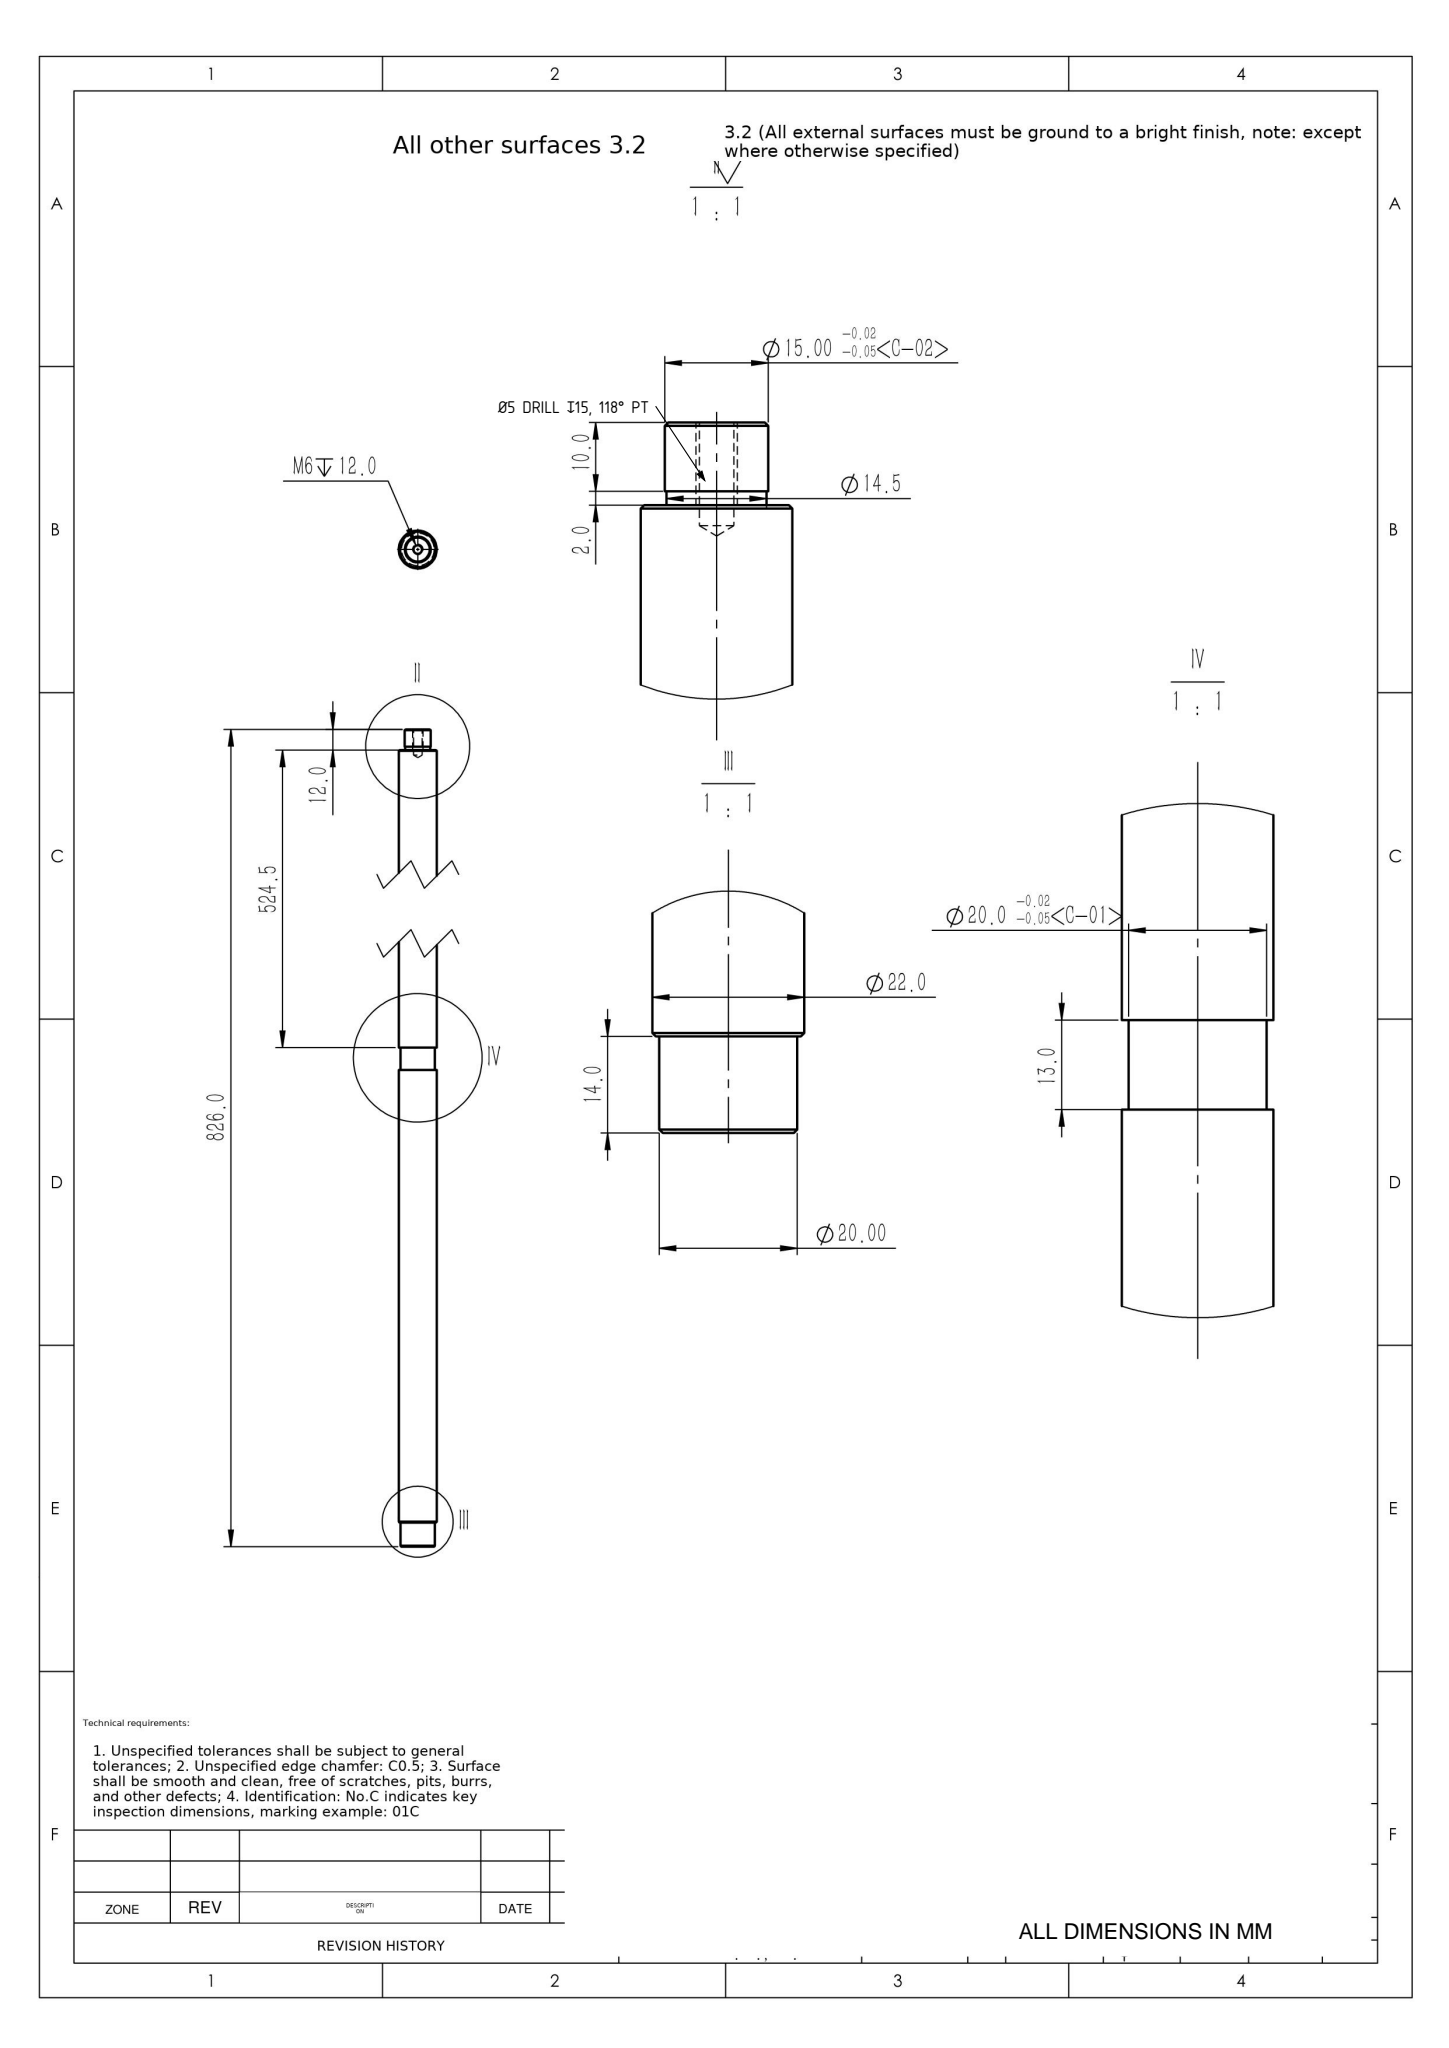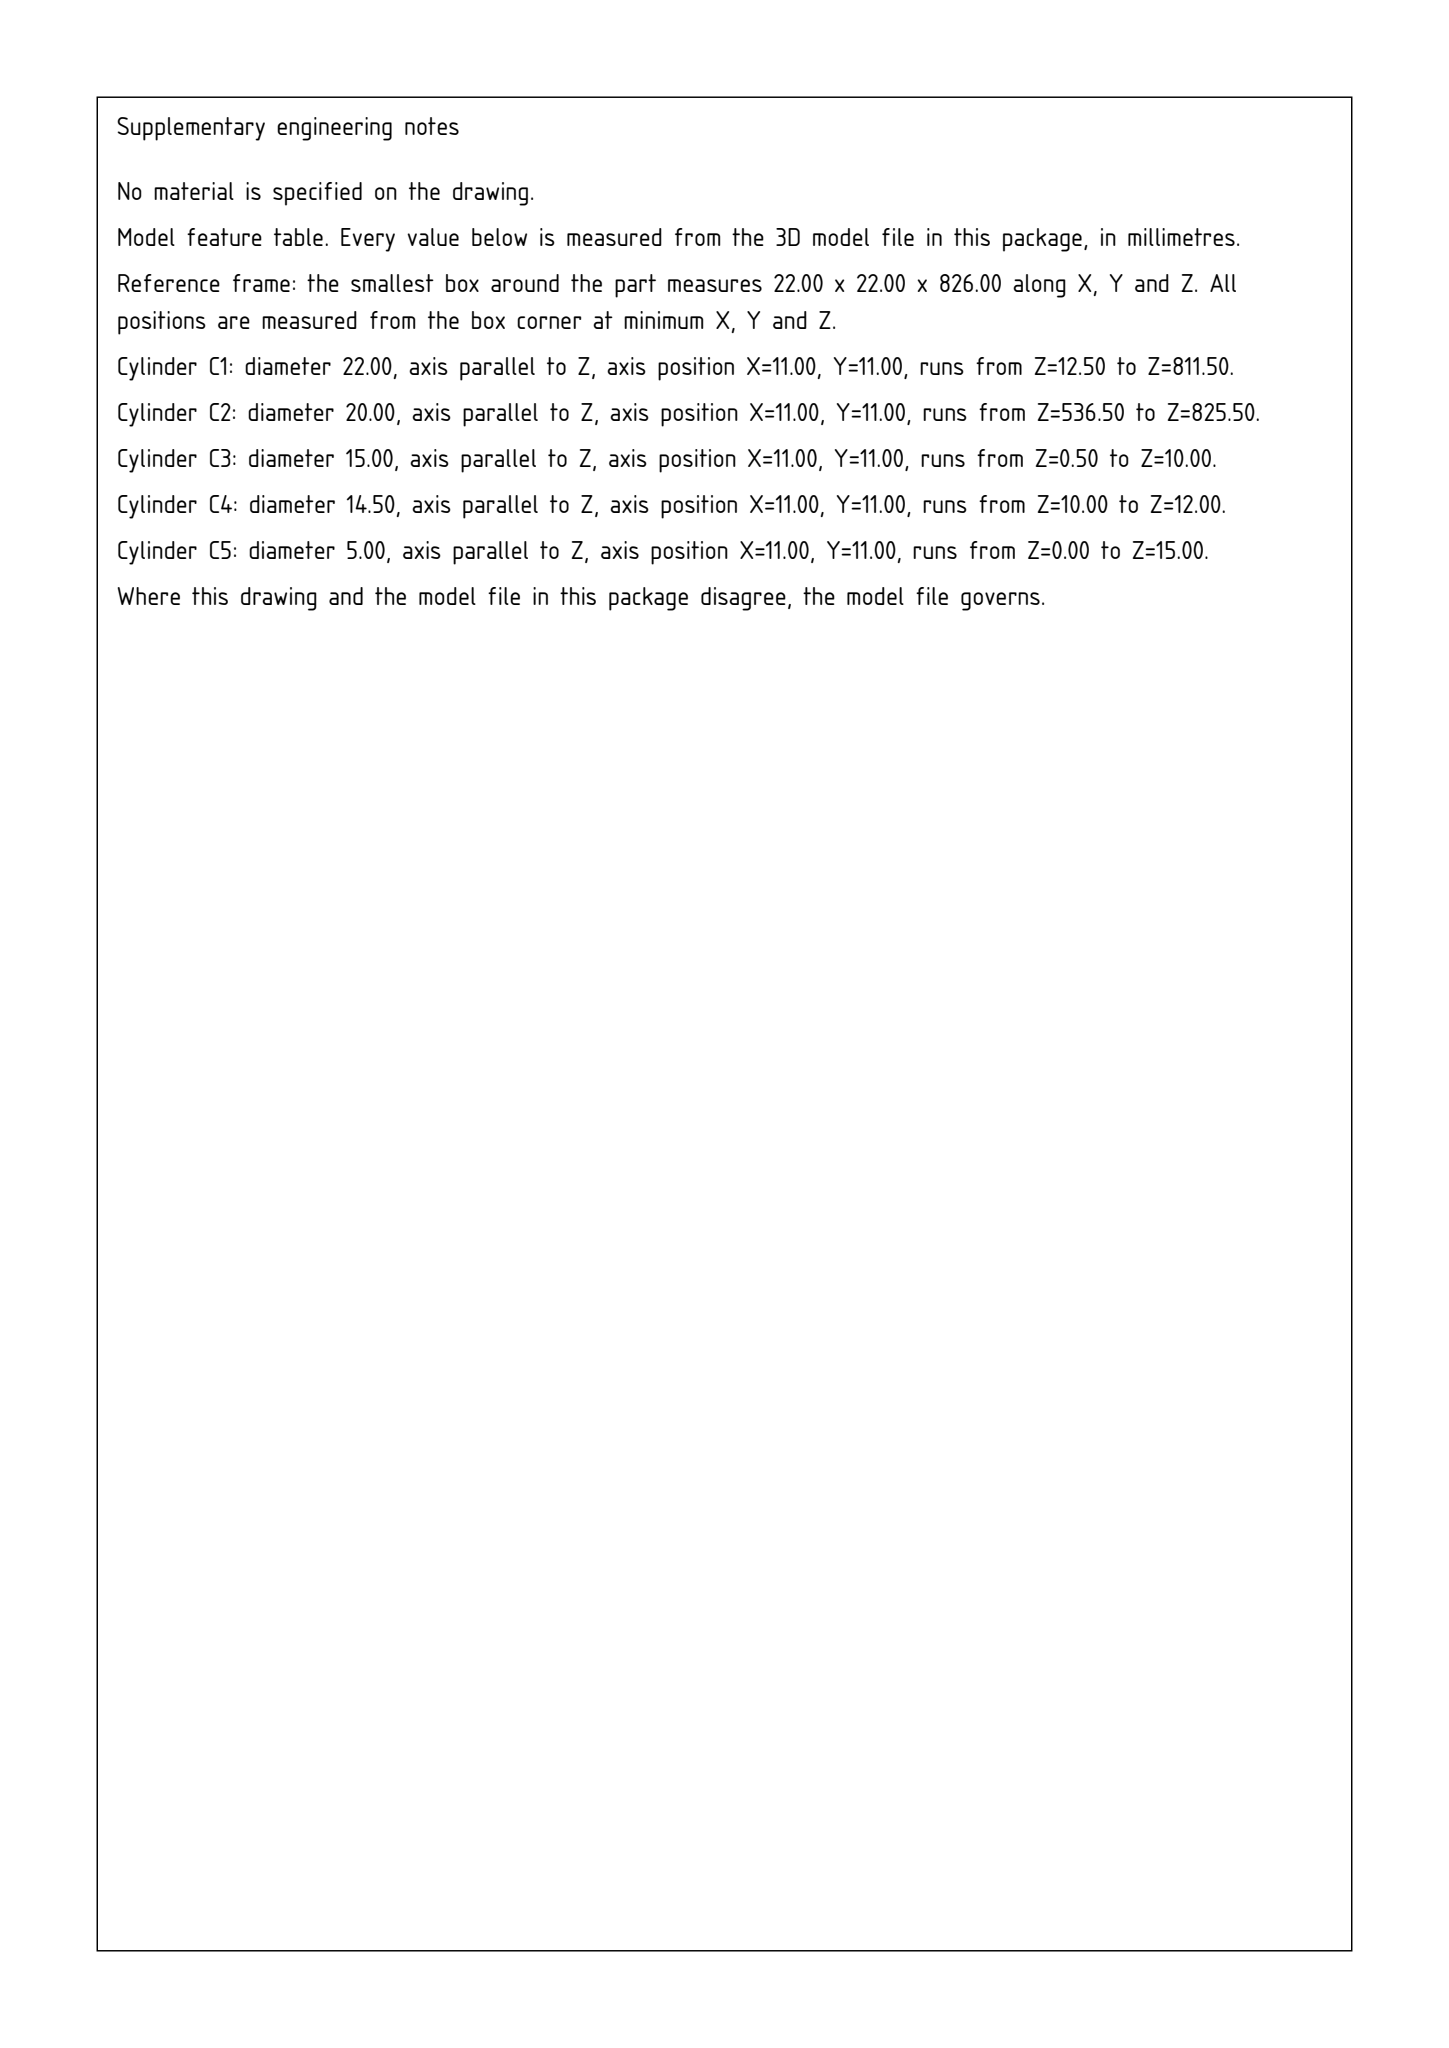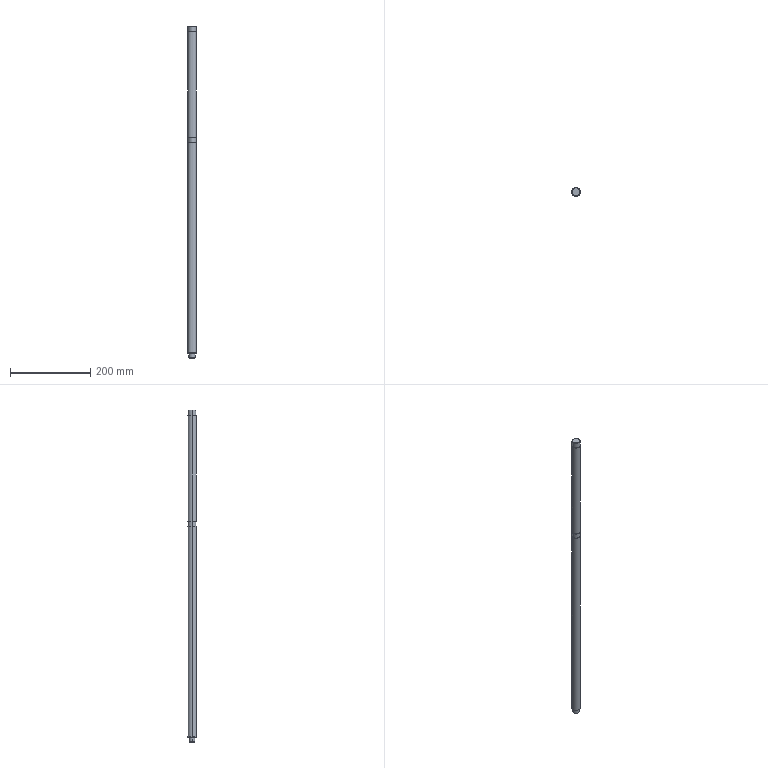Part | SolidWorks | mm | 1 solid | 31 faces | box 22 x 22 x 826 mm | volume 309409 mm3 | cylinder 14 | cone 10 | plane 7 | commonest cylinder face diameters 22 x4 20 x4 5 x2 15 x2 14.5 x2
Drawing notes:
VIEW II: Ø5 DRILL DP 15 (118° PT) BEFORE M6 DP 12.0 | from the solid: cylinder dia 5.0 along z, length 15.0 at (11,11); cone 118° ref dia 5.0
build123d program:
from build123d import *

# Parameters (mm, degrees)
SKETCH1_R             = 7.5
BOSS_EXTRUDE1_DEPTH   = 12
SKETCH2_R             = 11
BOSS_EXTRUDE2_DEPTH   = 800
SKETCH3_W             = 0.25
SKETCH3_H             = 2
CHAMFER1_SIZE         = 0.5
M6_TAPPED_HOLE1_D     = 5
M6_TAPPED_HOLE1_DEPTH = 15
M6_TAPPED_HOLE1_TIP   = 1.502
CHAMFER2_SIZE         = 0.5
SKETCH7_R             = 10
BOSS_EXTRUDE3_DEPTH   = 14
CHAMFER3_SIZE         = 0.5
SKETCH8_W             = 1
SKETCH8_H             = 13


with BuildPart() as part:
    # Sketch1 → Boss-Extrude1 (new body)
    with BuildSketch(Plane.XY):
        Circle(SKETCH1_R)
    extrude(amount=BOSS_EXTRUDE1_DEPTH)

    # Sketch2 → Boss-Extrude2 (add)
    with BuildSketch(Plane.XY.offset(12)):
        Circle(SKETCH2_R)
    extrude(amount=BOSS_EXTRUDE2_DEPTH)

    # Sketch3 → Cut-Revolve1 (revolve, cut)
    with BuildSketch(Plane(origin=(0, 0, 0), x_dir=(1, 0, 0), z_dir=(0, 1, 0))):
        with Locations((-7.375, -11)):
            Rectangle(SKETCH3_W, SKETCH3_H)
    revolve(axis=Axis((0, 0, 0), (0, 0, 1)), mode=Mode.SUBTRACT)

    # Chamfer1
    chamfer1_edges = [part.edges().sort_by_distance(p)[0] for p in [
        (-7.5, 0, 0),
    ]]
    chamfer(chamfer1_edges, length=CHAMFER1_SIZE)

    # M6 Tapped Hole1
    with Locations(Plane(origin=(0, 0, 0), x_dir=(-1, 0, 0), z_dir=(0, 0, -1))):
        with Locations((0, 0)):
            Hole(M6_TAPPED_HOLE1_D / 2, depth=M6_TAPPED_HOLE1_DEPTH)
            with Locations((0, 0, -(M6_TAPPED_HOLE1_DEPTH + M6_TAPPED_HOLE1_TIP / 2))):  # 118° drill point
                Cone(0, M6_TAPPED_HOLE1_D / 2, M6_TAPPED_HOLE1_TIP, mode=Mode.SUBTRACT)

    # Chamfer2
    chamfer2_edges = [part.edges().sort_by_distance(p)[0] for p in [
        (-11, 0, 12),
        (-11, 0, 812),
    ]]
    chamfer(chamfer2_edges, length=CHAMFER2_SIZE)

    # Sketch7 → Boss-Extrude3 (add)
    with BuildSketch(Plane.XY.offset(812)):
        Circle(SKETCH7_R)
    extrude(amount=BOSS_EXTRUDE3_DEPTH)

    # Chamfer3
    chamfer3_edges = [part.edges().sort_by_distance(p)[0] for p in [
        (-10, 0, 826),
    ]]
    chamfer(chamfer3_edges, length=CHAMFER3_SIZE)

    # Sketch8 → Cut-Revolve2 (revolve, cut)
    with BuildSketch(Plane(origin=(0, 0, 0), x_dir=(1, 0, 0), z_dir=(0, 1, 0))):
        with Locations((-10.5, -543)):
            Rectangle(SKETCH8_W, SKETCH8_H)
    revolve(axis=Axis((0, 0, 0), (0, 0, 1)), mode=Mode.SUBTRACT)


solid = part.part
STEP:
#1=CARTESIAN_POINT('',(-11.,0.,811.5));
#2=VERTEX_POINT('',#1);
#3=CARTESIAN_POINT('',(11.,0.,811.5));
#4=VERTEX_POINT('',#3);
#5=CARTESIAN_POINT('',(0.,0.,811.5));
#6=DIRECTION('',(0.,0.,-1.));
#7=DIRECTION('',(1.,0.,0.));
#8=AXIS2_PLACEMENT_3D('',#5,#6,#7);
#9=CIRCLE('',#8,11.);
#10=EDGE_CURVE('',#2,#4,#9,.T.);
#11=ORIENTED_EDGE('',*,*,#10,.T.);
#12=CARTESIAN_POINT('',(11.,0.,549.5));
#13=VERTEX_POINT('',#12);
#14=CARTESIAN_POINT('',(11.,0.,812.));
#15=DIRECTION('',(0.,0.,-1.));
#16=VECTOR('',#15,1000.);
#17=LINE('',#14,#16);
#18=EDGE_CURVE('',#4,#13,#17,.T.);
#19=ORIENTED_EDGE('',*,*,#18,.T.);
#20=CARTESIAN_POINT('',(-11.,0.,549.5));
#21=VERTEX_POINT('',#20);
#22=CARTESIAN_POINT('',(0.,0.,549.5));
#23=DIRECTION('',(0.,0.,-1.));
#24=DIRECTION('',(-1.,0.,0.));
#25=AXIS2_PLACEMENT_3D('',#22,#23,#24);
#26=CIRCLE('',#25,11.);
#27=EDGE_CURVE('',#21,#13,#26,.T.);
#28=ORIENTED_EDGE('',*,*,#27,.F.);
#29=CARTESIAN_POINT('',(-11.,0.,812.));
#30=DIRECTION('',(0.,0.,-1.));
#31=VECTOR('',#30,1000.);
#32=LINE('',#29,#31);
#33=EDGE_CURVE('',#2,#21,#32,.T.);
#34=ORIENTED_EDGE('',*,*,#33,.F.);
#35=EDGE_LOOP('',(#11,#19,#28,#34));
#36=FACE_OUTER_BOUND('',#35,.T.);
#37=CARTESIAN_POINT('',(0.,0.,812.));
#38=DIRECTION('',(0.,0.,-1.));
#39=DIRECTION('',(-1.,0.,0.));
#40=AXIS2_PLACEMENT_3D('',#37,#38,#39);
#41=CYLINDRICAL_SURFACE('',#40,11.);
#42=ADVANCED_FACE('',(#36),#41,.T.);
#43=CARTESIAN_POINT('',(10.5,0.,812.));
#44=VERTEX_POINT('',#43);
#45=CARTESIAN_POINT('',(-10.5,0.,812.));
#46=VERTEX_POINT('',#45);
#47=CARTESIAN_POINT('',(0.,0.,812.));
#48=DIRECTION('',(0.,0.,1.));
#49=DIRECTION('',(1.,0.,0.));
#50=AXIS2_PLACEMENT_3D('',#47,#48,#49);
#51=CIRCLE('',#50,10.5);
#52=EDGE_CURVE('',#44,#46,#51,.T.);
#53=ORIENTED_EDGE('',*,*,#52,.F.);
#54=CARTESIAN_POINT('',(10.5,0.,812.));
#55=DIRECTION('',(0.7071,0.,-0.7071));
#56=VECTOR('',#55,1000.);
#57=LINE('',#54,#56);
#58=EDGE_CURVE('',#44,#4,#57,.T.);
#59=ORIENTED_EDGE('',*,*,#58,.T.);
#60=ORIENTED_EDGE('',*,*,#10,.F.);
#61=CARTESIAN_POINT('',(-10.5,0.,812.));
#62=DIRECTION('',(-0.7071,0.,-0.7071));
#63=VECTOR('',#62,1000.);
#64=LINE('',#61,#63);
#65=EDGE_CURVE('',#46,#2,#64,.T.);
#66=ORIENTED_EDGE('',*,*,#65,.F.);
#67=EDGE_LOOP('',(#53,#59,#60,#66));
#68=FACE_OUTER_BOUND('',#67,.T.);
#69=CARTESIAN_POINT('',(0.,0.,812.));
#70=DIRECTION('',(0.,0.,-1.));
#71=DIRECTION('',(-1.,0.,0.));
#72=AXIS2_PLACEMENT_3D('',#69,#70,#71);
#73=CONICAL_SURFACE('',#72,10.5,0.7854);
#74=ADVANCED_FACE('',(#68),#73,.T.);
#75=CARTESIAN_POINT('',(-10.,0.,825.5));
#76=VERTEX_POINT('',#75);
#77=CARTESIAN_POINT('',(10.,0.,825.5));
#78=VERTEX_POINT('',#77);
#79=CARTESIAN_POINT('',(0.,0.,825.5));
#80=DIRECTION('',(0.,0.,-1.));
#81=DIRECTION('',(1.,0.,0.));
#82=AXIS2_PLACEMENT_3D('',#79,#80,#81);
#83=CIRCLE('',#82,10.);
#84=EDGE_CURVE('',#76,#78,#83,.T.);
#85=ORIENTED_EDGE('',*,*,#84,.T.);
#86=CARTESIAN_POINT('',(10.,0.,812.));
#87=VERTEX_POINT('',#86);
#88=CARTESIAN_POINT('',(10.,0.,826.));
#89=DIRECTION('',(0.,0.,-1.));
#90=VECTOR('',#89,1000.);
#91=LINE('',#88,#90);
#92=EDGE_CURVE('',#78,#87,#91,.T.);
#93=ORIENTED_EDGE('',*,*,#92,.T.);
#94=CARTESIAN_POINT('',(-10.,0.,812.));
#95=VERTEX_POINT('',#94);
#96=CARTESIAN_POINT('',(0.,0.,812.));
#97=DIRECTION('',(0.,0.,1.));
#98=DIRECTION('',(1.,0.,0.));
#99=AXIS2_PLACEMENT_3D('',#96,#97,#98);
#100=CIRCLE('',#99,10.);
#101=EDGE_CURVE('',#87,#95,#100,.T.);
#102=ORIENTED_EDGE('',*,*,#101,.T.);
#103=CARTESIAN_POINT('',(-10.,0.,826.));
#104=DIRECTION('',(0.,0.,-1.));
#105=VECTOR('',#104,1000.);
#106=LINE('',#103,#105);
#107=EDGE_CURVE('',#76,#95,#106,.T.);
#108=ORIENTED_EDGE('',*,*,#107,.F.);
#109=EDGE_LOOP('',(#85,#93,#102,#108));
#110=FACE_OUTER_BOUND('',#109,.T.);
#111=CARTESIAN_POINT('',(0.,0.,826.));
#112=DIRECTION('',(0.,0.,-1.));
#113=DIRECTION('',(-1.,0.,0.));
#114=AXIS2_PLACEMENT_3D('',#111,#112,#113);
#115=CYLINDRICAL_SURFACE('',#114,10.);
#116=ADVANCED_FACE('',(#110),#115,.T.);
#117=CARTESIAN_POINT('',(9.5,0.,826.));
#118=VERTEX_POINT('',#117);
#119=CARTESIAN_POINT('',(-9.5,0.,826.));
#120=VERTEX_POINT('',#119);
#121=CARTESIAN_POINT('',(0.,0.,826.));
#122=DIRECTION('',(0.,0.,1.));
#123=DIRECTION('',(1.,0.,0.));
#124=AXIS2_PLACEMENT_3D('',#121,#122,#123);
#125=CIRCLE('',#124,9.5);
#126=EDGE_CURVE('',#118,#120,#125,.T.);
#127=ORIENTED_EDGE('',*,*,#126,.F.);
#128=CARTESIAN_POINT('',(9.5,0.,826.));
#129=DIRECTION('',(0.7071,0.,-0.7071));
#130=VECTOR('',#129,1000.);
#131=LINE('',#128,#130);
#132=EDGE_CURVE('',#118,#78,#131,.T.);
#133=ORIENTED_EDGE('',*,*,#132,.T.);
#134=ORIENTED_EDGE('',*,*,#84,.F.);
#135=CARTESIAN_POINT('',(-9.5,0.,826.));
#136=DIRECTION('',(-0.7071,0.,-0.7071));
#137=VECTOR('',#136,1000.);
#138=LINE('',#135,#137);
#139=EDGE_CURVE('',#120,#76,#138,.T.);
#140=ORIENTED_EDGE('',*,*,#139,.F.);
#141=EDGE_LOOP('',(#127,#133,#134,#140));
#142=FACE_OUTER_BOUND('',#141,.T.);
#143=CARTESIAN_POINT('',(0.,0.,826.));
#144=DIRECTION('',(0.,0.,-1.));
#145=DIRECTION('',(-1.,0.,0.));
#146=AXIS2_PLACEMENT_3D('',#143,#144,#145);
#147=CONICAL_SURFACE('',#146,9.5,0.7854);
#148=ADVANCED_FACE('',(#142),#147,.T.);
#149=CARTESIAN_POINT('',(-10.,0.,549.5));
#150=VERTEX_POINT('',#149);
#151=CARTESIAN_POINT('',(10.,0.,549.5));
#152=VERTEX_POINT('',#151);
#153=CARTESIAN_POINT('',(0.,0.,549.5));
#154=DIRECTION('',(0.,0.,-1.));
#155=DIRECTION('',(-1.,0.,0.));
#156=AXIS2_PLACEMENT_3D('',#153,#154,#155);
#157=CIRCLE('',#156,10.);
#158=EDGE_CURVE('',#150,#152,#157,.T.);
#159=ORIENTED_EDGE('',*,*,#158,.T.);
#160=CARTESIAN_POINT('',(10.,0.,536.5));
#161=VERTEX_POINT('',#160);
#162=CARTESIAN_POINT('',(10.,0.,0.));
#163=DIRECTION('',(0.,0.,-1.));
#164=VECTOR('',#163,1000.);
#165=LINE('',#162,#164);
#166=EDGE_CURVE('',#152,#161,#165,.T.);
#167=ORIENTED_EDGE('',*,*,#166,.T.);
#168=CARTESIAN_POINT('',(-10.,0.,536.5));
#169=VERTEX_POINT('',#168);
#170=CARTESIAN_POINT('',(0.,0.,536.5));
#171=DIRECTION('',(0.,0.,-1.));
#172=DIRECTION('',(-1.,0.,0.));
#173=AXIS2_PLACEMENT_3D('',#170,#171,#172);
#174=CIRCLE('',#173,10.);
#175=EDGE_CURVE('',#169,#161,#174,.T.);
#176=ORIENTED_EDGE('',*,*,#175,.F.);
#177=CARTESIAN_POINT('',(-10.,0.,0.));
#178=DIRECTION('',(0.,0.,-1.));
#179=VECTOR('',#178,1000.);
#180=LINE('',#177,#179);
#181=EDGE_CURVE('',#150,#169,#180,.T.);
#182=ORIENTED_EDGE('',*,*,#181,.F.);
#183=EDGE_LOOP('',(#159,#167,#176,#182));
#184=FACE_OUTER_BOUND('',#183,.T.);
#185=CARTESIAN_POINT('',(0.,0.,0.));
#186=DIRECTION('',(0.,0.,-1.));
#187=DIRECTION('',(-1.,0.,0.));
#188=AXIS2_PLACEMENT_3D('',#185,#186,#187);
#189=CYLINDRICAL_SURFACE('',#188,10.);
#190=ADVANCED_FACE('',(#184),#189,.T.);
#191=CARTESIAN_POINT('',(-10.5,0.,12.));
#192=VERTEX_POINT('',#191);
#193=CARTESIAN_POINT('',(10.5,0.,12.));
#194=VERTEX_POINT('',#193);
#195=CARTESIAN_POINT('',(0.,0.,12.));
#196=DIRECTION('',(0.,0.,-1.));
#197=DIRECTION('',(1.,0.,0.));
#198=AXIS2_PLACEMENT_3D('',#195,#196,#197);
#199=CIRCLE('',#198,10.5);
#200=EDGE_CURVE('',#192,#194,#199,.T.);
#201=ORIENTED_EDGE('',*,*,#200,.F.);
#202=CARTESIAN_POINT('',(-11.,0.,12.5));
#203=VERTEX_POINT('',#202);
#204=CARTESIAN_POINT('',(-11.,0.,12.5));
#205=DIRECTION('',(-0.7071,0.,0.7071));
#206=VECTOR('',#205,1000.);
#207=LINE('',#204,#206);
#208=EDGE_CURVE('',#192,#203,#207,.T.);
#209=ORIENTED_EDGE('',*,*,#208,.T.);
#210=CARTESIAN_POINT('',(11.,0.,12.5));
#211=VERTEX_POINT('',#210);
#212=CARTESIAN_POINT('',(0.,0.,12.5));
#213=DIRECTION('',(0.,0.,1.));
#214=DIRECTION('',(1.,0.,0.));
#215=AXIS2_PLACEMENT_3D('',#212,#213,#214);
#216=CIRCLE('',#215,11.);
#217=EDGE_CURVE('',#211,#203,#216,.T.);
#218=ORIENTED_EDGE('',*,*,#217,.F.);
#219=CARTESIAN_POINT('',(11.,0.,12.5));
#220=DIRECTION('',(0.7071,0.,0.7071));
#221=VECTOR('',#220,1000.);
#222=LINE('',#219,#221);
#223=EDGE_CURVE('',#194,#211,#222,.T.);
#224=ORIENTED_EDGE('',*,*,#223,.F.);
#225=EDGE_LOOP('',(#201,#209,#218,#224));
#226=FACE_OUTER_BOUND('',#225,.T.);
#227=CARTESIAN_POINT('',(0.,0.,12.5));
#228=DIRECTION('',(0.,0.,1.));
#229=DIRECTION('',(1.,0.,0.));
#230=AXIS2_PLACEMENT_3D('',#227,#228,#229);
#231=CONICAL_SURFACE('',#230,11.,0.7854);
#232=ADVANCED_FACE('',(#226),#231,.T.);
#233=CARTESIAN_POINT('',(2.5,0.,15.));
#234=VERTEX_POINT('',#233);
#235=CARTESIAN_POINT('',(-2.5,0.,15.));
#236=VERTEX_POINT('',#235);
#237=CARTESIAN_POINT('',(0.,0.,15.));
#238=DIRECTION('',(0.,0.,-1.));
#239=DIRECTION('',(-1.,0.,0.));
#240=AXIS2_PLACEMENT_3D('',#237,#238,#239);
#241=CIRCLE('',#240,2.5);
#242=EDGE_CURVE('',#234,#236,#241,.T.);
#243=ORIENTED_EDGE('',*,*,#242,.F.);
#244=CARTESIAN_POINT('',(2.5,0.,-0.));
#245=VERTEX_POINT('',#244);
#246=CARTESIAN_POINT('',(2.5,0.,0.));
#247=DIRECTION('',(0.,0.,-1.));
#248=VECTOR('',#247,1000.);
#249=LINE('',#246,#248);
#250=EDGE_CURVE('',#234,#245,#249,.T.);
#251=ORIENTED_EDGE('',*,*,#250,.T.);
#252=CARTESIAN_POINT('',(-2.5,0.,-0.));
#253=VERTEX_POINT('',#252);
#254=CARTESIAN_POINT('',(0.,0.,-0.));
#255=DIRECTION('',(0.,0.,-1.));
#256=DIRECTION('',(-1.,0.,0.));
#257=AXIS2_PLACEMENT_3D('',#254,#255,#256);
#258=CIRCLE('',#257,2.5);
#259=EDGE_CURVE('',#245,#253,#258,.T.);
#260=ORIENTED_EDGE('',*,*,#259,.T.);
#261=CARTESIAN_POINT('',(-2.5,0.,0.));
#262=DIRECTION('',(0.,0.,-1.));
#263=VECTOR('',#262,1000.);
#264=LINE('',#261,#263);
#265=EDGE_CURVE('',#236,#253,#264,.T.);
#266=ORIENTED_EDGE('',*,*,#265,.F.);
#267=EDGE_LOOP('',(#243,#251,#260,#266));
#268=FACE_OUTER_BOUND('',#267,.T.);
#269=CARTESIAN_POINT('',(0.,0.,0.));
#270=DIRECTION('',(0.,0.,-1.));
#271=DIRECTION('',(-1.,0.,0.));
#272=AXIS2_PLACEMENT_3D('',#269,#270,#271);
#273=CYLINDRICAL_SURFACE('',#272,2.5);
#274=ADVANCED_FACE('',(#268),#273,.F.);
#275=CARTESIAN_POINT('',(-0.,0.,16.502));
#276=VERTEX_POINT('',#275);
#277=CARTESIAN_POINT('',(-2.5,0.,15.));
#278=DIRECTION('',(-0.8572,0.,-0.515));
#279=VECTOR('',#278,1000.);
#280=LINE('',#277,#279);
#281=EDGE_CURVE('',#276,#236,#280,.T.);
#282=ORIENTED_EDGE('',*,*,#281,.F.);
#283=CARTESIAN_POINT('',(2.5,0.,15.));
#284=DIRECTION('',(0.8572,0.,-0.515));
#285=VECTOR('',#284,1000.);
#286=LINE('',#283,#285);
#287=EDGE_CURVE('',#276,#234,#286,.T.);
#288=ORIENTED_EDGE('',*,*,#287,.T.);
#289=ORIENTED_EDGE('',*,*,#242,.T.);
#290=EDGE_LOOP('',(#282,#288,#289));
#291=FACE_OUTER_BOUND('',#290,.T.);
#292=CARTESIAN_POINT('',(0.,0.,15.));
#293=DIRECTION('',(0.,0.,-1.));
#294=DIRECTION('',(-1.,0.,0.));
#295=AXIS2_PLACEMENT_3D('',#292,#293,#294);
#296=CONICAL_SURFACE('',#295,2.5,1.03);
#297=ADVANCED_FACE('',(#291),#296,.F.);
#298=CARTESIAN_POINT('',(-7.,0.,0.));
#299=VERTEX_POINT('',#298);
#300=CARTESIAN_POINT('',(7.,0.,0.));
#301=VERTEX_POINT('',#300);
#302=CARTESIAN_POINT('',(0.,0.,0.));
#303=DIRECTION('',(0.,0.,-1.));
#304=DIRECTION('',(1.,0.,0.));
#305=AXIS2_PLACEMENT_3D('',#302,#303,#304);
#306=CIRCLE('',#305,7.);
#307=EDGE_CURVE('',#299,#301,#306,.T.);
#308=ORIENTED_EDGE('',*,*,#307,.F.);
#309=CARTESIAN_POINT('',(-7.5,0.,0.5));
#310=VERTEX_POINT('',#309);
#311=CARTESIAN_POINT('',(-7.5,0.,0.5));
#312=DIRECTION('',(-0.7071,0.,0.7071));
#313=VECTOR('',#312,1000.);
#314=LINE('',#311,#313);
#315=EDGE_CURVE('',#299,#310,#314,.T.);
#316=ORIENTED_EDGE('',*,*,#315,.T.);
#317=CARTESIAN_POINT('',(7.5,0.,0.5));
#318=VERTEX_POINT('',#317);
#319=CARTESIAN_POINT('',(0.,0.,0.5));
#320=DIRECTION('',(0.,0.,1.));
#321=DIRECTION('',(1.,0.,0.));
#322=AXIS2_PLACEMENT_3D('',#319,#320,#321);
#323=CIRCLE('',#322,7.5);
#324=EDGE_CURVE('',#318,#310,#323,.T.);
#325=ORIENTED_EDGE('',*,*,#324,.F.);
#326=CARTESIAN_POINT('',(7.5,0.,0.5));
#327=DIRECTION('',(0.7071,0.,0.7071));
#328=VECTOR('',#327,1000.);
#329=LINE('',#326,#328);
#330=EDGE_CURVE('',#301,#318,#329,.T.);
#331=ORIENTED_EDGE('',*,*,#330,.F.);
#332=EDGE_LOOP('',(#308,#316,#325,#331));
#333=FACE_OUTER_BOUND('',#332,.T.);
#334=CARTESIAN_POINT('',(0.,0.,0.5));
#335=DIRECTION('',(0.,0.,1.));
#336=DIRECTION('',(1.,0.,0.));
#337=AXIS2_PLACEMENT_3D('',#334,#335,#336);
#338=CONICAL_SURFACE('',#337,7.5,0.7854);
#339=ADVANCED_FACE('',(#333),#338,.T.);
#340=CARTESIAN_POINT('',(-7.5,0.,10.));
#341=VERTEX_POINT('',#340);
#342=CARTESIAN_POINT('',(7.5,0.,10.));
#343=VERTEX_POINT('',#342);
#344=CARTESIAN_POINT('',(0.,0.,10.));
#345=DIRECTION('',(0.,0.,-1.));
#346=DIRECTION('',(-1.,0.,0.));
#347=AXIS2_PLACEMENT_3D('',#344,#345,#346);
#348=CIRCLE('',#347,7.5);
#349=EDGE_CURVE('',#341,#343,#348,.T.);
#350=ORIENTED_EDGE('',*,*,#349,.T.);
#351=CARTESIAN_POINT('',(7.5,0.,12.));
#352=DIRECTION('',(0.,0.,-1.));
#353=VECTOR('',#352,1000.);
#354=LINE('',#351,#353);
#355=EDGE_CURVE('',#343,#318,#354,.T.);
#356=ORIENTED_EDGE('',*,*,#355,.T.);
#357=ORIENTED_EDGE('',*,*,#324,.T.);
#358=CARTESIAN_POINT('',(-7.5,0.,12.));
#359=DIRECTION('',(0.,0.,-1.));
#360=VECTOR('',#359,1000.);
#361=LINE('',#358,#360);
#362=EDGE_CURVE('',#341,#310,#361,.T.);
#363=ORIENTED_EDGE('',*,*,#362,.F.);
#364=EDGE_LOOP('',(#350,#356,#357,#363));
#365=FACE_OUTER_BOUND('',#364,.T.);
#366=CARTESIAN_POINT('',(0.,0.,12.));
#367=DIRECTION('',(0.,0.,-1.));
#368=DIRECTION('',(-1.,0.,0.));
#369=AXIS2_PLACEMENT_3D('',#366,#367,#368);
#370=CYLINDRICAL_SURFACE('',#369,7.5);
#371=ADVANCED_FACE('',(#365),#370,.T.);
#372=CARTESIAN_POINT('',(-7.25,0.,12.));
#373=VERTEX_POINT('',#372);
#374=CARTESIAN_POINT('',(7.25,0.,12.));
#375=VERTEX_POINT('',#374);
#376=CARTESIAN_POINT('',(0.,0.,12.));
#377=DIRECTION('',(0.,0.,-1.));
#378=DIRECTION('',(-1.,0.,0.));
#379=AXIS2_PLACEMENT_3D('',#376,#377,#378);
#380=CIRCLE('',#379,7.25);
#381=EDGE_CURVE('',#373,#375,#380,.T.);
#382=ORIENTED_EDGE('',*,*,#381,.T.);
#383=CARTESIAN_POINT('',(7.25,0.,10.));
#384=VERTEX_POINT('',#383);
#385=CARTESIAN_POINT('',(7.25,0.,0.));
#386=DIRECTION('',(0.,0.,-1.));
#387=VECTOR('',#386,1000.);
#388=LINE('',#385,#387);
#389=EDGE_CURVE('',#375,#384,#388,.T.);
#390=ORIENTED_EDGE('',*,*,#389,.T.);
#391=CARTESIAN_POINT('',(-7.25,0.,10.));
#392=VERTEX_POINT('',#391);
#393=CARTESIAN_POINT('',(0.,0.,10.));
#394=DIRECTION('',(0.,0.,-1.));
#395=DIRECTION('',(-1.,0.,0.));
#396=AXIS2_PLACEMENT_3D('',#393,#394,#395);
#397=CIRCLE('',#396,7.25);
#398=EDGE_CURVE('',#392,#384,#397,.T.);
#399=ORIENTED_EDGE('',*,*,#398,.F.);
#400=CARTESIAN_POINT('',(-7.25,0.,0.));
#401=DIRECTION('',(0.,0.,-1.));
#402=VECTOR('',#401,1000.);
#403=LINE('',#400,#402);
#404=EDGE_CURVE('',#373,#392,#403,.T.);
#405=ORIENTED_EDGE('',*,*,#404,.F.);
#406=EDGE_LOOP('',(#382,#390,#399,#405));
#407=FACE_OUTER_BOUND('',#406,.T.);
#408=CARTESIAN_POINT('',(0.,0.,0.));
#409=DIRECTION('',(0.,0.,-1.));
#410=DIRECTION('',(-1.,0.,0.));
#411=AXIS2_PLACEMENT_3D('',#408,#409,#410);
#412=CYLINDRICAL_SURFACE('',#411,7.25);
#413=ADVANCED_FACE('',(#407),#412,.T.);
#414=CARTESIAN_POINT('',(-11.,0.,536.5));
#415=VERTEX_POINT('',#414);
#416=CARTESIAN_POINT('',(11.,0.,536.5));
#417=VERTEX_POINT('',#416);
#418=CARTESIAN_POINT('',(0.,0.,536.5));
#419=DIRECTION('',(0.,0.,-1.));
#420=DIRECTION('',(-1.,0.,0.));
#421=AXIS2_PLACEMENT_3D('',#418,#419,#420);
#422=CIRCLE('',#421,11.);
#423=EDGE_CURVE('',#415,#417,#422,.T.);
#424=ORIENTED_EDGE('',*,*,#423,.T.);
#425=CARTESIAN_POINT('',(11.,0.,812.));
#426=DIRECTION('',(0.,0.,-1.));
#427=VECTOR('',#426,1000.);
#428=LINE('',#425,#427);
#429=EDGE_CURVE('',#417,#211,#428,.T.);
#430=ORIENTED_EDGE('',*,*,#429,.T.);
#431=ORIENTED_EDGE('',*,*,#217,.T.);
#432=CARTESIAN_POINT('',(-11.,0.,812.));
#433=DIRECTION('',(0.,0.,-1.));
#434=VECTOR('',#433,1000.);
#435=LINE('',#432,#434);
#436=EDGE_CURVE('',#415,#203,#435,.T.);
#437=ORIENTED_EDGE('',*,*,#436,.F.);
#438=EDGE_LOOP('',(#424,#430,#431,#437));
#439=FACE_OUTER_BOUND('',#438,.T.);
#440=CARTESIAN_POINT('',(0.,0.,812.));
#441=DIRECTION('',(0.,0.,-1.));
#442=DIRECTION('',(-1.,0.,0.));
#443=AXIS2_PLACEMENT_3D('',#440,#441,#442);
#444=CYLINDRICAL_SURFACE('',#443,11.);
#445=ADVANCED_FACE('',(#439),#444,.T.);
#446=ORIENTED_EDGE('',*,*,#429,.F.);
#447=CARTESIAN_POINT('',(0.,0.,536.5));
#448=DIRECTION('',(0.,0.,-1.));
#449=DIRECTION('',(-1.,0.,0.));
#450=AXIS2_PLACEMENT_3D('',#447,#448,#449);
#451=CIRCLE('',#450,11.);
#452=EDGE_CURVE('',#417,#415,#451,.T.);
#453=ORIENTED_EDGE('',*,*,#452,.T.);
#454=ORIENTED_EDGE('',*,*,#436,.T.);
#455=CARTESIAN_POINT('',(0.,0.,12.5));
#456=DIRECTION('',(0.,0.,1.));
#457=DIRECTION('',(1.,0.,0.));
#458=AXIS2_PLACEMENT_3D('',#455,#456,#457);
#459=CIRCLE('',#458,11.);
#460=EDGE_CURVE('',#203,#211,#459,.T.);
#461=ORIENTED_EDGE('',*,*,#460,.T.);
#462=EDGE_LOOP('',(#446,#453,#454,#461));
#463=FACE_OUTER_BOUND('',#462,.T.);
#464=CARTESIAN_POINT('',(0.,0.,812.));
#465=DIRECTION('',(0.,0.,-1.));
#466=DIRECTION('',(-1.,0.,0.));
#467=AXIS2_PLACEMENT_3D('',#464,#465,#466);
#468=CYLINDRICAL_SURFACE('',#467,11.);
#469=ADVANCED_FACE('',(#463),#468,.T.);
#470=CARTESIAN_POINT('',(0.,0.,12.));
#471=DIRECTION('',(0.,0.,-1.));
#472=DIRECTION('',(1.,0.,0.));
#473=AXIS2_PLACEMENT_3D('',#470,#471,#472);
#474=CIRCLE('',#473,10.5);
#475=EDGE_CURVE('',#194,#192,#474,.T.);
#476=ORIENTED_EDGE('',*,*,#475,.T.);
#477=ORIENTED_EDGE('',*,*,#200,.T.);
#478=EDGE_LOOP('',(#476,#477));
#479=FACE_OUTER_BOUND('',#478,.T.);
#480=ORIENTED_EDGE('',*,*,#381,.F.);
#481=CARTESIAN_POINT('',(0.,0.,12.));
#482=DIRECTION('',(0.,0.,-1.));
#483=DIRECTION('',(-1.,0.,0.));
#484=AXIS2_PLACEMENT_3D('',#481,#482,#483);
#485=CIRCLE('',#484,7.25);
#486=EDGE_CURVE('',#375,#373,#485,.T.);
#487=ORIENTED_EDGE('',*,*,#486,.F.);
#488=EDGE_LOOP('',(#480,#487));
#489=FACE_BOUND('',#488,.T.);
#490=CARTESIAN_POINT('',(0.,0.,12.));
#491=DIRECTION('',(0.,0.,1.));
#492=DIRECTION('',(1.,0.,0.));
#493=AXIS2_PLACEMENT_3D('',#490,#491,#492);
#494=PLANE('',#493);
#495=ADVANCED_FACE('',(#479,#489),#494,.F.);
#496=ORIENTED_EDGE('',*,*,#349,.F.);
#497=CARTESIAN_POINT('',(0.,0.,10.));
#498=DIRECTION('',(0.,0.,-1.));
#499=DIRECTION('',(-1.,0.,0.));
#500=AXIS2_PLACEMENT_3D('',#497,#498,#499);
#501=CIRCLE('',#500,7.5);
#502=EDGE_CURVE('',#343,#341,#501,.T.);
#503=ORIENTED_EDGE('',*,*,#502,.F.);
#504=EDGE_LOOP('',(#496,#503));
#505=FACE_OUTER_BOUND('',#504,.T.);
#506=ORIENTED_EDGE('',*,*,#398,.T.);
#507=CARTESIAN_POINT('',(0.,0.,10.));
#508=DIRECTION('',(0.,0.,-1.));
#509=DIRECTION('',(-1.,0.,0.));
#510=AXIS2_PLACEMENT_3D('',#507,#508,#509);
#511=CIRCLE('',#510,7.25);
#512=EDGE_CURVE('',#384,#392,#511,.T.);
#513=ORIENTED_EDGE('',*,*,#512,.T.);
#514=EDGE_LOOP('',(#506,#513));
#515=FACE_BOUND('',#514,.T.);
#516=CARTESIAN_POINT('',(-7.5,0.,10.));
#517=DIRECTION('',(0.,0.,-1.));
#518=DIRECTION('',(-1.,0.,0.));
#519=AXIS2_PLACEMENT_3D('',#516,#517,#518);
#520=PLANE('',#519);
#521=ADVANCED_FACE('',(#505,#515),#520,.F.);
#522=ORIENTED_EDGE('',*,*,#389,.F.);
#523=ORIENTED_EDGE('',*,*,#486,.T.);
#524=ORIENTED_EDGE('',*,*,#404,.T.);
#525=ORIENTED_EDGE('',*,*,#512,.F.);
#526=EDGE_LOOP('',(#522,#523,#524,#525));
#527=FACE_OUTER_BOUND('',#526,.T.);
#528=CARTESIAN_POINT('',(0.,0.,0.));
#529=DIRECTION('',(0.,0.,-1.));
#530=DIRECTION('',(-1.,0.,0.));
#531=AXIS2_PLACEMENT_3D('',#528,#529,#530);
#532=CYLINDRICAL_SURFACE('',#531,7.25);
#533=ADVANCED_FACE('',(#527),#532,.T.);
#534=CARTESIAN_POINT('',(0.,0.,-0.));
#535=DIRECTION('',(0.,0.,-1.));
#536=DIRECTION('',(-1.,0.,0.));
#537=AXIS2_PLACEMENT_3D('',#534,#535,#536);
#538=CIRCLE('',#537,2.5);
#539=EDGE_CURVE('',#253,#245,#538,.T.);
#540=ORIENTED_EDGE('',*,*,#539,.F.);
#541=ORIENTED_EDGE('',*,*,#259,.F.);
#542=EDGE_LOOP('',(#540,#541));
#543=FACE_BOUND('',#542,.T.);
#544=CARTESIAN_POINT('',(0.,0.,0.));
#545=DIRECTION('',(0.,0.,-1.));
#546=DIRECTION('',(1.,0.,0.));
#547=AXIS2_PLACEMENT_3D('',#544,#545,#546);
#548=CIRCLE('',#547,7.);
#549=EDGE_CURVE('',#301,#299,#548,.T.);
#550=ORIENTED_EDGE('',*,*,#549,.T.);
#551=ORIENTED_EDGE('',*,*,#307,.T.);
#552=EDGE_LOOP('',(#550,#551));
#553=FACE_OUTER_BOUND('',#552,.T.);
#554=CARTESIAN_POINT('',(0.,0.,0.));
#555=DIRECTION('',(0.,0.,1.));
#556=DIRECTION('',(1.,0.,0.));
#557=AXIS2_PLACEMENT_3D('',#554,#555,#556);
#558=PLANE('',#557);
#559=ADVANCED_FACE('',(#543,#553),#558,.F.);
#560=ORIENTED_EDGE('',*,*,#355,.F.);
#561=ORIENTED_EDGE('',*,*,#502,.T.);
#562=ORIENTED_EDGE('',*,*,#362,.T.);
#563=CARTESIAN_POINT('',(0.,0.,0.5));
#564=DIRECTION('',(0.,0.,1.));
#565=DIRECTION('',(1.,0.,0.));
#566=AXIS2_PLACEMENT_3D('',#563,#564,#565);
#567=CIRCLE('',#566,7.5);
#568=EDGE_CURVE('',#310,#318,#567,.T.);
#569=ORIENTED_EDGE('',*,*,#568,.T.);
#570=EDGE_LOOP('',(#560,#561,#562,#569));
#571=FACE_OUTER_BOUND('',#570,.T.);
#572=CARTESIAN_POINT('',(0.,0.,12.));
#573=DIRECTION('',(0.,0.,-1.));
#574=DIRECTION('',(-1.,0.,0.));
#575=AXIS2_PLACEMENT_3D('',#572,#573,#574);
#576=CYLINDRICAL_SURFACE('',#575,7.5);
#577=ADVANCED_FACE('',(#571),#576,.T.);
#578=ORIENTED_EDGE('',*,*,#315,.F.);
#579=ORIENTED_EDGE('',*,*,#549,.F.);
#580=ORIENTED_EDGE('',*,*,#330,.T.);
#581=ORIENTED_EDGE('',*,*,#568,.F.);
#582=EDGE_LOOP('',(#578,#579,#580,#581));
#583=FACE_OUTER_BOUND('',#582,.T.);
#584=CARTESIAN_POINT('',(0.,0.,0.5));
#585=DIRECTION('',(0.,0.,1.));
#586=DIRECTION('',(1.,0.,0.));
#587=AXIS2_PLACEMENT_3D('',#584,#585,#586);
#588=CONICAL_SURFACE('',#587,7.5,0.7854);
#589=ADVANCED_FACE('',(#583),#588,.T.);
#590=ORIENTED_EDGE('',*,*,#287,.F.);
#591=ORIENTED_EDGE('',*,*,#281,.T.);
#592=CARTESIAN_POINT('',(0.,0.,15.));
#593=DIRECTION('',(0.,0.,-1.));
#594=DIRECTION('',(-1.,0.,0.));
#595=AXIS2_PLACEMENT_3D('',#592,#593,#594);
#596=CIRCLE('',#595,2.5);
#597=EDGE_CURVE('',#236,#234,#596,.T.);
#598=ORIENTED_EDGE('',*,*,#597,.T.);
#599=EDGE_LOOP('',(#590,#591,#598));
#600=FACE_OUTER_BOUND('',#599,.T.);
#601=CARTESIAN_POINT('',(0.,0.,15.));
#602=DIRECTION('',(0.,0.,-1.));
#603=DIRECTION('',(-1.,0.,0.));
#604=AXIS2_PLACEMENT_3D('',#601,#602,#603);
#605=CONICAL_SURFACE('',#604,2.5,1.03);
#606=ADVANCED_FACE('',(#600),#605,.F.);
#607=ORIENTED_EDGE('',*,*,#250,.F.);
#608=ORIENTED_EDGE('',*,*,#597,.F.);
#609=ORIENTED_EDGE('',*,*,#265,.T.);
#610=ORIENTED_EDGE('',*,*,#539,.T.);
#611=EDGE_LOOP('',(#607,#608,#609,#610));
#612=FACE_OUTER_BOUND('',#611,.T.);
#613=CARTESIAN_POINT('',(0.,0.,0.));
#614=DIRECTION('',(0.,0.,-1.));
#615=DIRECTION('',(-1.,0.,0.));
#616=AXIS2_PLACEMENT_3D('',#613,#614,#615);
#617=CYLINDRICAL_SURFACE('',#616,2.5);
#618=ADVANCED_FACE('',(#612),#617,.F.);
#619=ORIENTED_EDGE('',*,*,#208,.F.);
#620=ORIENTED_EDGE('',*,*,#475,.F.);
#621=ORIENTED_EDGE('',*,*,#223,.T.);
#622=ORIENTED_EDGE('',*,*,#460,.F.);
#623=EDGE_LOOP('',(#619,#620,#621,#622));
#624=FACE_OUTER_BOUND('',#623,.T.);
#625=CARTESIAN_POINT('',(0.,0.,12.5));
#626=DIRECTION('',(0.,0.,1.));
#627=DIRECTION('',(1.,0.,0.));
#628=AXIS2_PLACEMENT_3D('',#625,#626,#627);
#629=CONICAL_SURFACE('',#628,11.,0.7854);
#630=ADVANCED_FACE('',(#624),#629,.T.);
#631=ORIENTED_EDGE('',*,*,#158,.F.);
#632=CARTESIAN_POINT('',(0.,0.,549.5));
#633=DIRECTION('',(0.,0.,-1.));
#634=DIRECTION('',(-1.,0.,0.));
#635=AXIS2_PLACEMENT_3D('',#632,#633,#634);
#636=CIRCLE('',#635,10.);
#637=EDGE_CURVE('',#152,#150,#636,.T.);
#638=ORIENTED_EDGE('',*,*,#637,.F.);
#639=EDGE_LOOP('',(#631,#638));
#640=FACE_BOUND('',#639,.T.);
#641=ORIENTED_EDGE('',*,*,#27,.T.);
#642=CARTESIAN_POINT('',(0.,0.,549.5));
#643=DIRECTION('',(0.,0.,-1.));
#644=DIRECTION('',(-1.,0.,0.));
#645=AXIS2_PLACEMENT_3D('',#642,#643,#644);
#646=CIRCLE('',#645,11.);
#647=EDGE_CURVE('',#13,#21,#646,.T.);
#648=ORIENTED_EDGE('',*,*,#647,.T.);
#649=EDGE_LOOP('',(#641,#648));
#650=FACE_OUTER_BOUND('',#649,.T.);
#651=CARTESIAN_POINT('',(-11.,0.,549.5));
#652=DIRECTION('',(0.,0.,1.));
#653=DIRECTION('',(1.,0.,0.));
#654=AXIS2_PLACEMENT_3D('',#651,#652,#653);
#655=PLANE('',#654);
#656=ADVANCED_FACE('',(#640,#650),#655,.F.);
#657=ORIENTED_EDGE('',*,*,#166,.F.);
#658=ORIENTED_EDGE('',*,*,#637,.T.);
#659=ORIENTED_EDGE('',*,*,#181,.T.);
#660=CARTESIAN_POINT('',(0.,0.,536.5));
#661=DIRECTION('',(0.,0.,-1.));
#662=DIRECTION('',(-1.,0.,0.));
#663=AXIS2_PLACEMENT_3D('',#660,#661,#662);
#664=CIRCLE('',#663,10.);
#665=EDGE_CURVE('',#161,#169,#664,.T.);
#666=ORIENTED_EDGE('',*,*,#665,.F.);
#667=EDGE_LOOP('',(#657,#658,#659,#666));
#668=FACE_OUTER_BOUND('',#667,.T.);
#669=CARTESIAN_POINT('',(0.,0.,0.));
#670=DIRECTION('',(0.,0.,-1.));
#671=DIRECTION('',(-1.,0.,0.));
#672=AXIS2_PLACEMENT_3D('',#669,#670,#671);
#673=CYLINDRICAL_SURFACE('',#672,10.);
#674=ADVANCED_FACE('',(#668),#673,.T.);
#675=ORIENTED_EDGE('',*,*,#423,.F.);
#676=ORIENTED_EDGE('',*,*,#452,.F.);
#677=EDGE_LOOP('',(#675,#676));
#678=FACE_OUTER_BOUND('',#677,.T.);
#679=ORIENTED_EDGE('',*,*,#175,.T.);
#680=ORIENTED_EDGE('',*,*,#665,.T.);
#681=EDGE_LOOP('',(#679,#680));
#682=FACE_BOUND('',#681,.T.);
#683=CARTESIAN_POINT('',(-11.,0.,536.5));
#684=DIRECTION('',(0.,0.,-1.));
#685=DIRECTION('',(-1.,0.,0.));
#686=AXIS2_PLACEMENT_3D('',#683,#684,#685);
#687=PLANE('',#686);
#688=ADVANCED_FACE('',(#678,#682),#687,.F.);
#689=CARTESIAN_POINT('',(0.,0.,826.));
#690=DIRECTION('',(0.,0.,1.));
#691=DIRECTION('',(1.,0.,0.));
#692=AXIS2_PLACEMENT_3D('',#689,#690,#691);
#693=CIRCLE('',#692,9.5);
#694=EDGE_CURVE('',#120,#118,#693,.T.);
#695=ORIENTED_EDGE('',*,*,#694,.T.);
#696=ORIENTED_EDGE('',*,*,#126,.T.);
#697=EDGE_LOOP('',(#695,#696));
#698=FACE_OUTER_BOUND('',#697,.T.);
#699=CARTESIAN_POINT('',(0.,0.,826.));
#700=DIRECTION('',(0.,0.,1.));
#701=DIRECTION('',(1.,0.,0.));
#702=AXIS2_PLACEMENT_3D('',#699,#700,#701);
#703=PLANE('',#702);
#704=ADVANCED_FACE('',(#698),#703,.T.);
#705=ORIENTED_EDGE('',*,*,#132,.F.);
#706=ORIENTED_EDGE('',*,*,#694,.F.);
#707=ORIENTED_EDGE('',*,*,#139,.T.);
#708=CARTESIAN_POINT('',(0.,0.,825.5));
#709=DIRECTION('',(0.,0.,-1.));
#710=DIRECTION('',(1.,0.,0.));
#711=AXIS2_PLACEMENT_3D('',#708,#709,#710);
#712=CIRCLE('',#711,10.);
#713=EDGE_CURVE('',#78,#76,#712,.T.);
#714=ORIENTED_EDGE('',*,*,#713,.F.);
#715=EDGE_LOOP('',(#705,#706,#707,#714));
#716=FACE_OUTER_BOUND('',#715,.T.);
#717=CARTESIAN_POINT('',(0.,0.,826.));
#718=DIRECTION('',(0.,0.,-1.));
#719=DIRECTION('',(-1.,0.,0.));
#720=AXIS2_PLACEMENT_3D('',#717,#718,#719);
#721=CONICAL_SURFACE('',#720,9.5,0.7854);
#722=ADVANCED_FACE('',(#716),#721,.T.);
#723=ORIENTED_EDGE('',*,*,#92,.F.);
#724=ORIENTED_EDGE('',*,*,#713,.T.);
#725=ORIENTED_EDGE('',*,*,#107,.T.);
#726=CARTESIAN_POINT('',(0.,0.,812.));
#727=DIRECTION('',(0.,0.,1.));
#728=DIRECTION('',(1.,0.,0.));
#729=AXIS2_PLACEMENT_3D('',#726,#727,#728);
#730=CIRCLE('',#729,10.);
#731=EDGE_CURVE('',#95,#87,#730,.T.);
#732=ORIENTED_EDGE('',*,*,#731,.T.);
#733=EDGE_LOOP('',(#723,#724,#725,#732));
#734=FACE_OUTER_BOUND('',#733,.T.);
#735=CARTESIAN_POINT('',(0.,0.,826.));
#736=DIRECTION('',(0.,0.,-1.));
#737=DIRECTION('',(-1.,0.,0.));
#738=AXIS2_PLACEMENT_3D('',#735,#736,#737);
#739=CYLINDRICAL_SURFACE('',#738,10.);
#740=ADVANCED_FACE('',(#734),#739,.T.);
#741=ORIENTED_EDGE('',*,*,#731,.F.);
#742=ORIENTED_EDGE('',*,*,#101,.F.);
#743=EDGE_LOOP('',(#741,#742));
#744=FACE_BOUND('',#743,.T.);
#745=CARTESIAN_POINT('',(0.,0.,812.));
#746=DIRECTION('',(0.,0.,1.));
#747=DIRECTION('',(1.,0.,0.));
#748=AXIS2_PLACEMENT_3D('',#745,#746,#747);
#749=CIRCLE('',#748,10.5);
#750=EDGE_CURVE('',#46,#44,#749,.T.);
#751=ORIENTED_EDGE('',*,*,#750,.T.);
#752=ORIENTED_EDGE('',*,*,#52,.T.);
#753=EDGE_LOOP('',(#751,#752));
#754=FACE_OUTER_BOUND('',#753,.T.);
#755=CARTESIAN_POINT('',(0.,0.,812.));
#756=DIRECTION('',(0.,0.,1.));
#757=DIRECTION('',(1.,0.,0.));
#758=AXIS2_PLACEMENT_3D('',#755,#756,#757);
#759=PLANE('',#758);
#760=ADVANCED_FACE('',(#744,#754),#759,.T.);
#761=ORIENTED_EDGE('',*,*,#58,.F.);
#762=ORIENTED_EDGE('',*,*,#750,.F.);
#763=ORIENTED_EDGE('',*,*,#65,.T.);
#764=CARTESIAN_POINT('',(0.,0.,811.5));
#765=DIRECTION('',(0.,0.,-1.));
#766=DIRECTION('',(1.,0.,0.));
#767=AXIS2_PLACEMENT_3D('',#764,#765,#766);
#768=CIRCLE('',#767,11.);
#769=EDGE_CURVE('',#4,#2,#768,.T.);
#770=ORIENTED_EDGE('',*,*,#769,.F.);
#771=EDGE_LOOP('',(#761,#762,#763,#770));
#772=FACE_OUTER_BOUND('',#771,.T.);
#773=CARTESIAN_POINT('',(0.,0.,812.));
#774=DIRECTION('',(0.,0.,-1.));
#775=DIRECTION('',(-1.,0.,0.));
#776=AXIS2_PLACEMENT_3D('',#773,#774,#775);
#777=CONICAL_SURFACE('',#776,10.5,0.7854);
#778=ADVANCED_FACE('',(#772),#777,.T.);
#779=ORIENTED_EDGE('',*,*,#18,.F.);
#780=ORIENTED_EDGE('',*,*,#769,.T.);
#781=ORIENTED_EDGE('',*,*,#33,.T.);
#782=ORIENTED_EDGE('',*,*,#647,.F.);
#783=EDGE_LOOP('',(#779,#780,#781,#782));
#784=FACE_OUTER_BOUND('',#783,.T.);
#785=CARTESIAN_POINT('',(0.,0.,812.));
#786=DIRECTION('',(0.,0.,-1.));
#787=DIRECTION('',(-1.,0.,0.));
#788=AXIS2_PLACEMENT_3D('',#785,#786,#787);
#789=CYLINDRICAL_SURFACE('',#788,11.);
#790=ADVANCED_FACE('',(#784),#789,.T.);
#791=CLOSED_SHELL('',(#42,#74,#116,#148,#190,#232,#274,#297,#339,#371,#413,#445,#469,#495,#521,#533,#559,#577,#589,#606,#618,#630,#656,#674,#688,#704,#722,#740,#760,#778,#790));
#792=MANIFOLD_SOLID_BREP('',#791);
#793=CARTESIAN_POINT('',(0.,0.,0.));
#794=DIRECTION('',(0.,0.,1.));
#795=DIRECTION('',(1.,0.,0.));
#796=AXIS2_PLACEMENT_3D('',#793,#794,#795);
#797=(LENGTH_UNIT()NAMED_UNIT(*)SI_UNIT(.MILLI.,.METRE.));
#798=UNCERTAINTY_MEASURE_WITH_UNIT(LENGTH_MEASURE(0.00001),#797,'','');
#799=(NAMED_UNIT(*)PLANE_ANGLE_UNIT()SI_UNIT($,.RADIAN.));
#800=(NAMED_UNIT(*)SI_UNIT($,.STERADIAN.)SOLID_ANGLE_UNIT());
#801=(GEOMETRIC_REPRESENTATION_CONTEXT(3)GLOBAL_UNCERTAINTY_ASSIGNED_CONTEXT((#798))GLOBAL_UNIT_ASSIGNED_CONTEXT((#797,#799,#800))REPRESENTATION_CONTEXT('',''));
#802=ADVANCED_BREP_SHAPE_REPRESENTATION('',(#792,#796),#801);